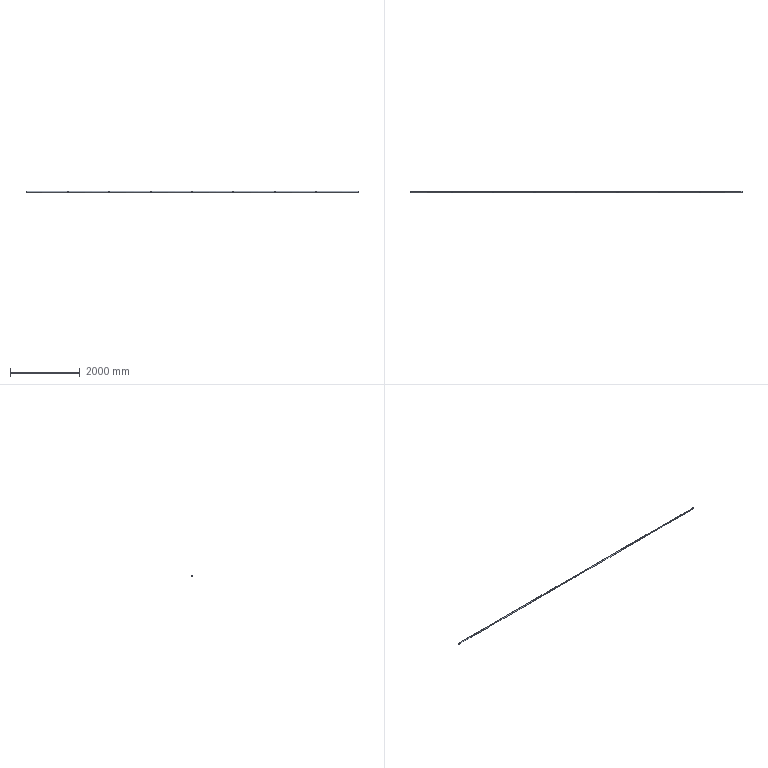Component | SolidWorks | PlatformGuardrail3-2 | 8 solids | 48 faces | volume 2691653 mm3 | cylinder 46 | plane 2 | commonest cylinder face diameters 33.5 x16 27.5 x16 33.6 x14 | material Plain Carbon Steel